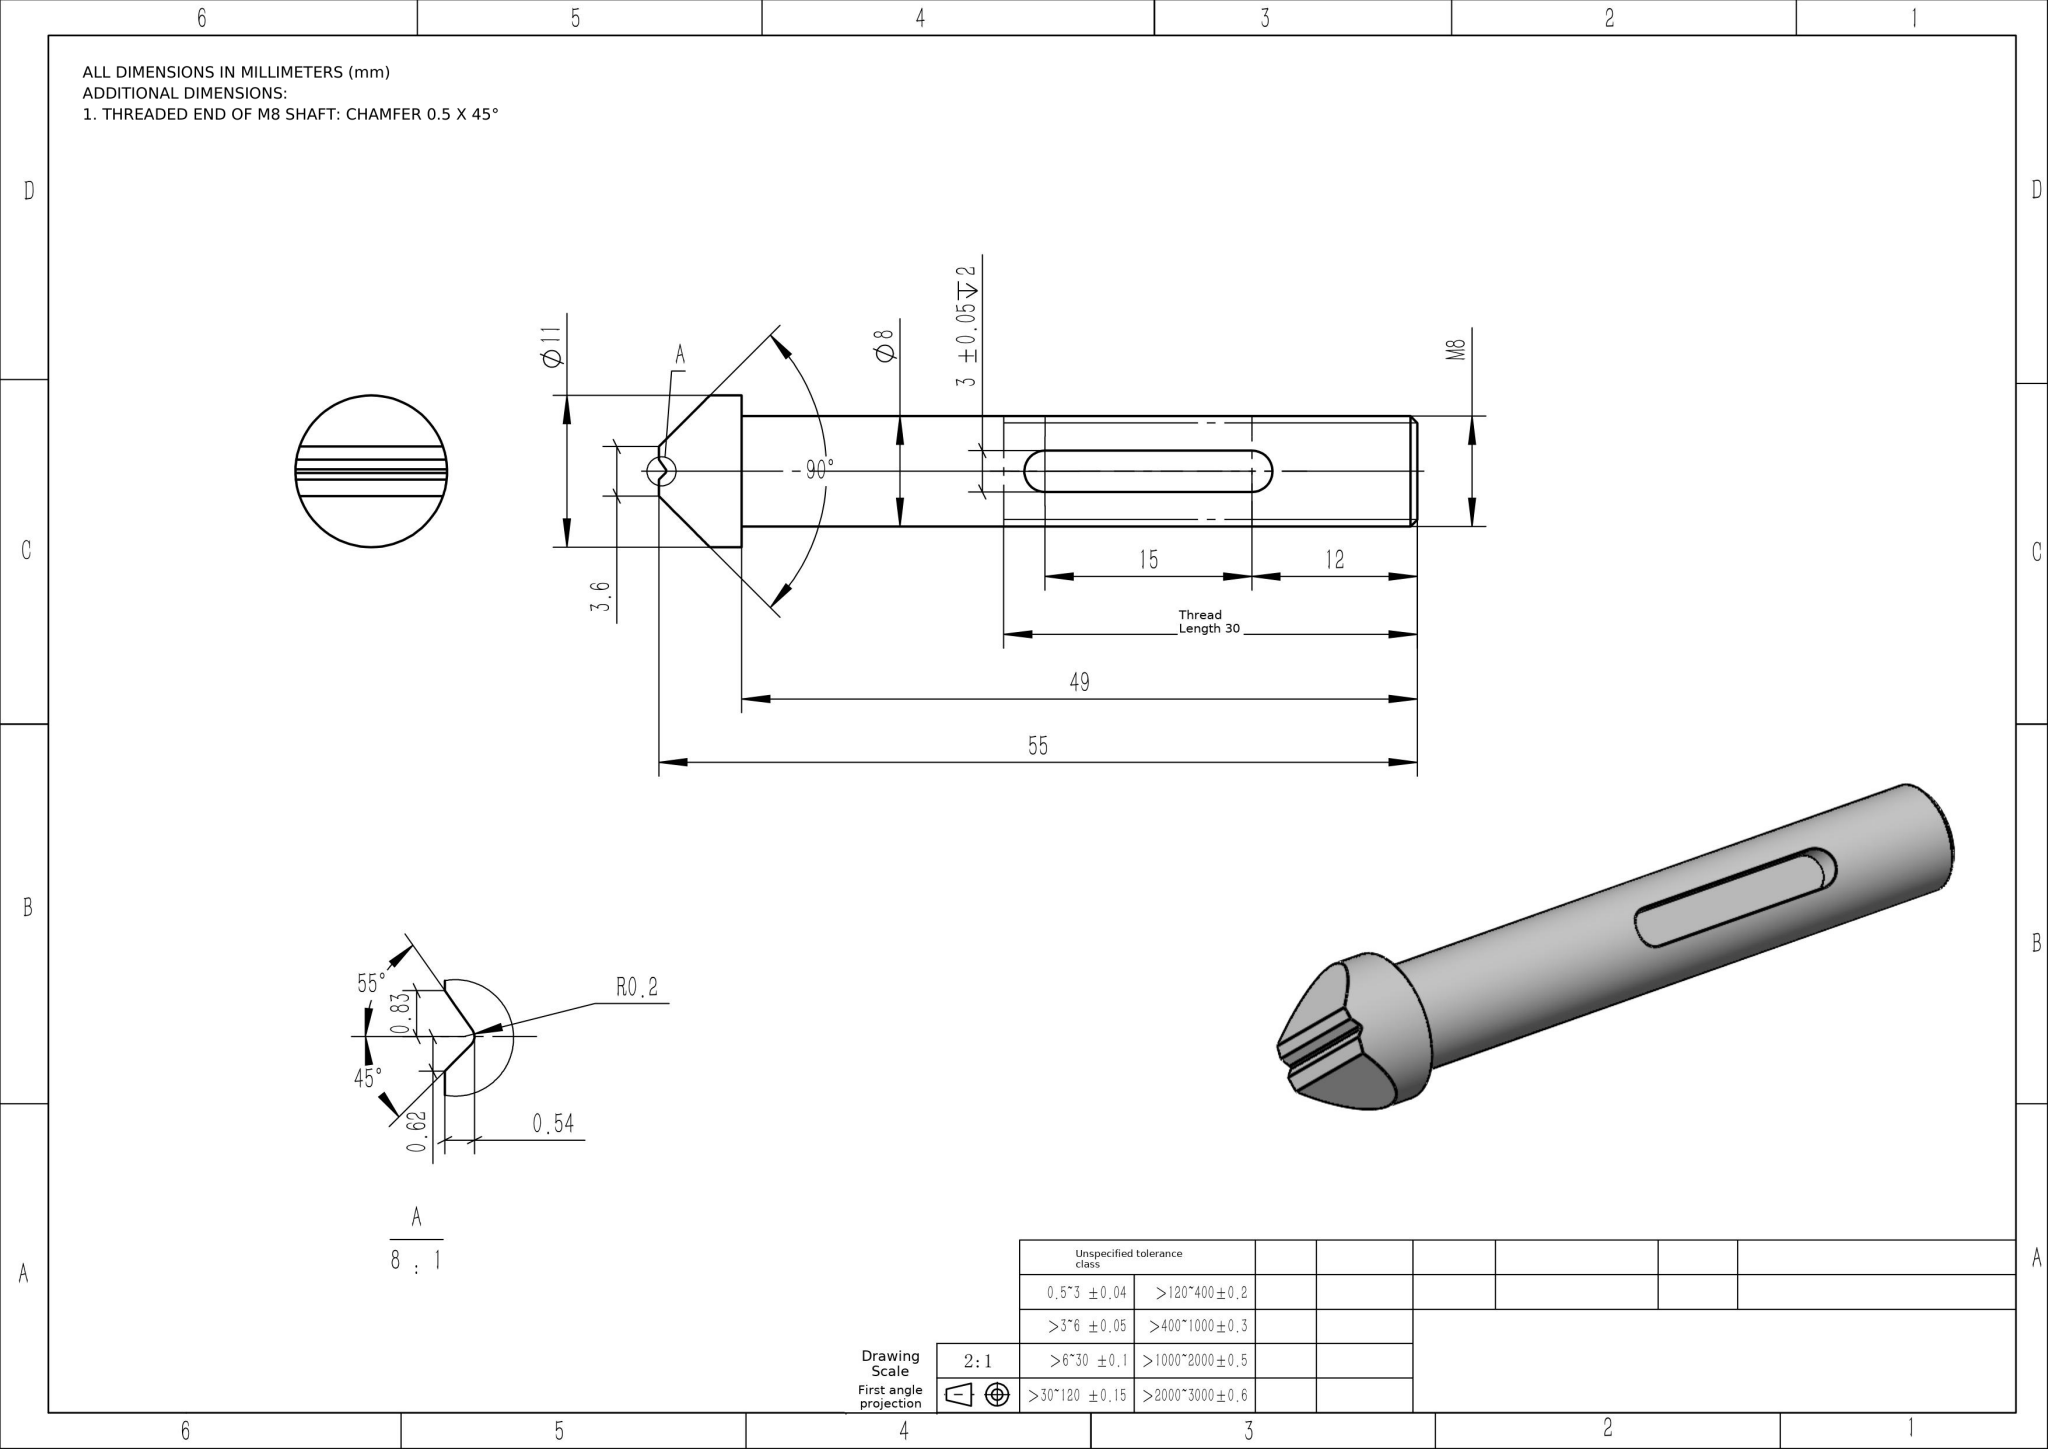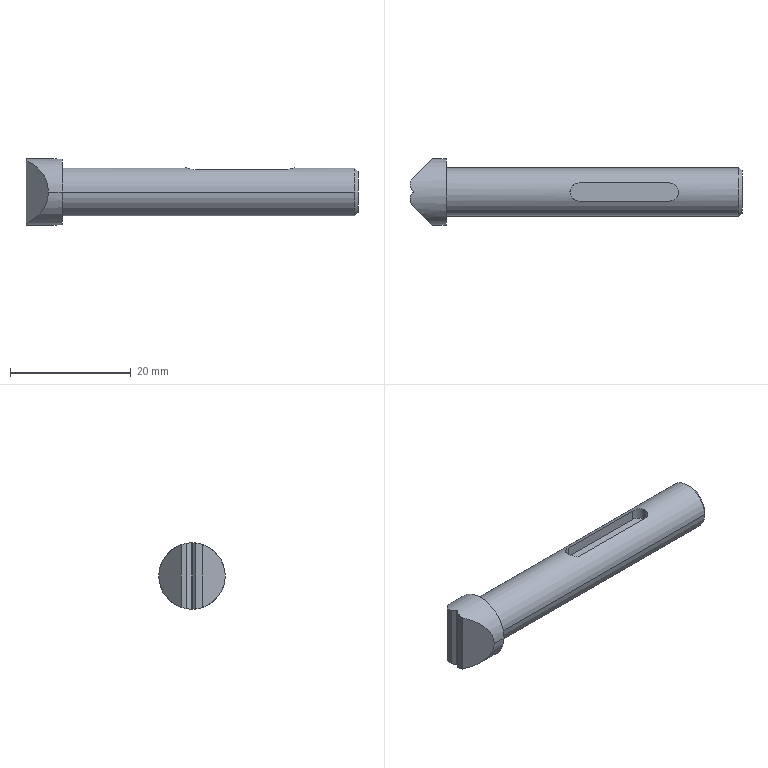Part | NX | mm | 1 solid | 22 faces | box 55 x 11 x 11 mm | volume 2840 mm3 | plane 11 | cylinder 9 | cone 2 | commonest cylinder face diameters 3 x3 0.4 x2 8 x2 11 x2
STEP:
#1=COLOUR_RGB('',0.698,0.698,0.698);
#2=FILL_AREA_STYLE_COLOUR('',#1);
#3=FILL_AREA_STYLE('',(#2));
#4=SURFACE_STYLE_FILL_AREA(#3);
#5=SURFACE_SIDE_STYLE('',(#4));
#6=SURFACE_STYLE_USAGE(.BOTH.,#5);
#7=PRESENTATION_STYLE_ASSIGNMENT((#6));
#8=CARTESIAN_POINT('',(44.5,0.,2.));
#9=VERTEX_POINT('',#8);
#10=CARTESIAN_POINT('',(43.,1.5,2.));
#11=VERTEX_POINT('',#10);
#12=CARTESIAN_POINT('',(43.,0.,2.));
#13=DIRECTION('',(0.,0.,1.));
#14=DIRECTION('',(1.,0.,0.));
#15=AXIS2_PLACEMENT_3D('',#12,#13,#14);
#16=CIRCLE('',#15,1.5);
#17=EDGE_CURVE('',#9,#11,#16,.T.);
#18=ORIENTED_EDGE('',*,*,#17,.F.);
#19=CARTESIAN_POINT('',(44.5,0.,4.));
#20=VERTEX_POINT('',#19);
#21=CARTESIAN_POINT('',(44.5,0.,2.));
#22=DIRECTION('',(0.,0.,1.));
#23=VECTOR('',#22,1000.);
#24=LINE('',#21,#23);
#25=EDGE_CURVE('',#9,#20,#24,.T.);
#26=ORIENTED_EDGE('',*,*,#25,.T.);
#27=CARTESIAN_POINT('',(43.,1.5,3.708));
#28=VERTEX_POINT('',#27);
#29=CARTESIAN_POINT('',(44.5,0.,4.));
#30=CARTESIAN_POINT('',(44.5,0.0988,4.));
#31=CARTESIAN_POINT('',(44.49,0.1991,3.996));
#32=CARTESIAN_POINT('',(44.451,0.3921,3.982));
#33=CARTESIAN_POINT('',(44.423,0.486,3.971));
#34=CARTESIAN_POINT('',(44.346,0.6687,3.945));
#35=CARTESIAN_POINT('',(44.3,0.7547,3.929));
#36=CARTESIAN_POINT('',(44.192,0.9162,3.895));
#37=CARTESIAN_POINT('',(44.129,0.9924,3.876));
#38=CARTESIAN_POINT('',(43.991,1.13,3.838));
#39=CARTESIAN_POINT('',(43.917,1.191,3.819));
#40=CARTESIAN_POINT('',(43.755,1.3,3.783));
#41=CARTESIAN_POINT('',(43.668,1.347,3.767));
#42=CARTESIAN_POINT('',(43.398,1.459,3.725));
#43=CARTESIAN_POINT('',(43.2,1.5,3.708));
#44=CARTESIAN_POINT('',(43.,1.5,3.708));
#45=B_SPLINE_CURVE_WITH_KNOTS('',3,(#29,#30,#31,#32,#33,#34,#35,#36,#37,#38,#39,#40,#41,#42,#43,#44),.UNSPECIFIED.,.F.,.F.,(4,2,2,2,2,2,2,4),(0.002367,0.002663,0.002958,0.003254,0.003549,0.003845,0.00414,0.004731),.UNSPECIFIED.);
#46=EDGE_CURVE('',#20,#28,#45,.T.);
#47=ORIENTED_EDGE('',*,*,#46,.T.);
#48=CARTESIAN_POINT('',(43.,1.5,2.));
#49=DIRECTION('',(0.,0.,1.));
#50=VECTOR('',#49,1000.);
#51=LINE('',#48,#50);
#52=EDGE_CURVE('',#11,#28,#51,.T.);
#53=ORIENTED_EDGE('',*,*,#52,.F.);
#54=EDGE_LOOP('',(#18,#26,#47,#53));
#55=FACE_OUTER_BOUND('',#54,.T.);
#56=CARTESIAN_POINT('',(43.,0.,2.));
#57=DIRECTION('',(0.,0.,1.));
#58=DIRECTION('',(1.,0.,0.));
#59=AXIS2_PLACEMENT_3D('',#56,#57,#58);
#60=CYLINDRICAL_SURFACE('',#59,1.5);
#61=ADVANCED_FACE('',(#55),#60,.F.);
#62=CARTESIAN_POINT('',(0.5037,0.1375,-5.498));
#63=VERTEX_POINT('',#62);
#64=CARTESIAN_POINT('',(0.5399,0.02275,-5.5));
#65=VERTEX_POINT('',#64);
#66=CARTESIAN_POINT('',(0.5037,0.1375,-5.498));
#67=CARTESIAN_POINT('',(0.5273,0.1038,-5.499));
#68=CARTESIAN_POINT('',(0.5399,0.06353,-5.5));
#69=CARTESIAN_POINT('',(0.5399,0.02275,-5.5));
#70=B_SPLINE_CURVE_WITH_KNOTS('',3,(#66,#67,#68,#69),.UNSPECIFIED.,.F.,.F.,(4,4),(0.,0.0001217),.UNSPECIFIED.);
#71=EDGE_CURVE('',#63,#65,#70,.T.);
#72=ORIENTED_EDGE('',*,*,#71,.T.);
#73=CARTESIAN_POINT('',(0.5399,0.02275,5.5));
#74=VERTEX_POINT('',#73);
#75=CARTESIAN_POINT('',(0.5399,0.02275,-10.));
#76=DIRECTION('',(0.,0.,1.));
#77=VECTOR('',#76,1000.);
#78=LINE('',#75,#77);
#79=EDGE_CURVE('',#65,#74,#78,.T.);
#80=ORIENTED_EDGE('',*,*,#79,.T.);
#81=CARTESIAN_POINT('',(0.5037,0.1375,5.498));
#82=VERTEX_POINT('',#81);
#83=CARTESIAN_POINT('',(0.5399,0.02275,5.5));
#84=CARTESIAN_POINT('',(0.5399,0.06334,5.5));
#85=CARTESIAN_POINT('',(0.5273,0.1038,5.499));
#86=CARTESIAN_POINT('',(0.5037,0.1375,5.498));
#87=B_SPLINE_CURVE_WITH_KNOTS('',3,(#83,#84,#85,#86),.UNSPECIFIED.,.F.,.F.,(4,4),(0.0001563,0.0002779),.UNSPECIFIED.);
#88=EDGE_CURVE('',#74,#82,#87,.T.);
#89=ORIENTED_EDGE('',*,*,#88,.T.);
#90=CARTESIAN_POINT('',(0.5037,0.1375,-10.));
#91=DIRECTION('',(0.,0.,1.));
#92=VECTOR('',#91,1000.);
#93=LINE('',#90,#92);
#94=EDGE_CURVE('',#63,#82,#93,.T.);
#95=ORIENTED_EDGE('',*,*,#94,.F.);
#96=EDGE_LOOP('',(#72,#80,#89,#95));
#97=FACE_OUTER_BOUND('',#96,.T.);
#98=CARTESIAN_POINT('',(0.3399,0.02275,-10.));
#99=DIRECTION('',(0.,0.,1.));
#100=DIRECTION('',(1.,0.,0.));
#101=AXIS2_PLACEMENT_3D('',#98,#99,#100);
#102=CYLINDRICAL_SURFACE('',#101,0.2);
#103=ADVANCED_FACE('',(#97),#102,.F.);
#104=CARTESIAN_POINT('',(55.,3.5,0.));
#105=VERTEX_POINT('',#104);
#106=CARTESIAN_POINT('',(55.,-3.5,0.));
#107=VERTEX_POINT('',#106);
#108=CARTESIAN_POINT('',(55.,-0.,0.));
#109=DIRECTION('',(1.,-0.,0.));
#110=DIRECTION('',(0.,1.,0.));
#111=AXIS2_PLACEMENT_3D('',#108,#109,#110);
#112=CIRCLE('',#111,3.5);
#113=EDGE_CURVE('',#105,#107,#112,.T.);
#114=ORIENTED_EDGE('',*,*,#113,.F.);
#115=CARTESIAN_POINT('',(54.5,4.,0.));
#116=VERTEX_POINT('',#115);
#117=CARTESIAN_POINT('',(55.,3.5,0.));
#118=DIRECTION('',(-0.7071,0.7071,0.));
#119=VECTOR('',#118,1000.);
#120=LINE('',#117,#119);
#121=EDGE_CURVE('',#105,#116,#120,.T.);
#122=ORIENTED_EDGE('',*,*,#121,.T.);
#123=CARTESIAN_POINT('',(54.5,-4.,0.));
#124=VERTEX_POINT('',#123);
#125=CARTESIAN_POINT('',(54.5,-0.,0.));
#126=DIRECTION('',(1.,-0.,0.));
#127=DIRECTION('',(0.,1.,0.));
#128=AXIS2_PLACEMENT_3D('',#125,#126,#127);
#129=CIRCLE('',#128,4.);
#130=EDGE_CURVE('',#116,#124,#129,.T.);
#131=ORIENTED_EDGE('',*,*,#130,.T.);
#132=CARTESIAN_POINT('',(55.,-3.5,0.));
#133=DIRECTION('',(-0.7071,-0.7071,0.));
#134=VECTOR('',#133,1000.);
#135=LINE('',#132,#134);
#136=EDGE_CURVE('',#107,#124,#135,.T.);
#137=ORIENTED_EDGE('',*,*,#136,.F.);
#138=EDGE_LOOP('',(#114,#122,#131,#137));
#139=FACE_OUTER_BOUND('',#138,.T.);
#140=CARTESIAN_POINT('',(55.,-0.,0.));
#141=DIRECTION('',(-1.,0.,0.));
#142=DIRECTION('',(0.,-1.,0.));
#143=AXIS2_PLACEMENT_3D('',#140,#141,#142);
#144=CONICAL_SURFACE('',#143,3.5,0.7854);
#145=ADVANCED_FACE('',(#139),#144,.T.);
#146=CARTESIAN_POINT('',(43.,-1.5,3.708));
#147=VERTEX_POINT('',#146);
#148=CARTESIAN_POINT('',(43.,-1.5,3.708));
#149=CARTESIAN_POINT('',(43.1,-1.5,3.708));
#150=CARTESIAN_POINT('',(43.198,-1.49,3.712));
#151=CARTESIAN_POINT('',(43.391,-1.451,3.727));
#152=CARTESIAN_POINT('',(43.487,-1.422,3.739));
#153=CARTESIAN_POINT('',(43.759,-1.309,3.781));
#154=CARTESIAN_POINT('',(43.924,-1.197,3.819));
#155=CARTESIAN_POINT('',(44.198,-0.9232,3.895));
#156=CARTESIAN_POINT('',(44.309,-0.7573,3.932));
#157=CARTESIAN_POINT('',(44.422,-0.4867,3.971));
#158=CARTESIAN_POINT('',(44.451,-0.3912,3.982));
#159=CARTESIAN_POINT('',(44.49,-0.197,3.996));
#160=CARTESIAN_POINT('',(44.5,-0.09895,4.));
#161=CARTESIAN_POINT('',(44.5,0.,4.));
#162=B_SPLINE_CURVE_WITH_KNOTS('',3,(#148,#149,#150,#151,#152,#153,#154,#155,#156,#157,#158,#159,#160,#161),.UNSPECIFIED.,.F.,.F.,(4,2,2,2,2,2,4),(0.,0.0002959,0.0005918,0.001184,0.001775,0.002071,0.002367),.UNSPECIFIED.);
#163=EDGE_CURVE('',#147,#20,#162,.T.);
#164=ORIENTED_EDGE('',*,*,#163,.F.);
#165=CARTESIAN_POINT('',(28.,-1.5,3.708));
#166=VERTEX_POINT('',#165);
#167=CARTESIAN_POINT('',(55.,-1.5,3.708));
#168=DIRECTION('',(1.,-0.,0.));
#169=VECTOR('',#168,1000.);
#170=LINE('',#167,#169);
#171=EDGE_CURVE('',#166,#147,#170,.T.);
#172=ORIENTED_EDGE('',*,*,#171,.F.);
#173=CARTESIAN_POINT('',(28.,1.5,3.708));
#174=VERTEX_POINT('',#173);
#175=CARTESIAN_POINT('',(28.,1.5,3.708));
#176=CARTESIAN_POINT('',(27.9,1.5,3.708));
#177=CARTESIAN_POINT('',(27.802,1.49,3.712));
#178=CARTESIAN_POINT('',(27.609,1.451,3.727));
#179=CARTESIAN_POINT('',(27.513,1.422,3.739));
#180=CARTESIAN_POINT('',(27.242,1.309,3.781));
#181=CARTESIAN_POINT('',(27.077,1.198,3.819));
#182=CARTESIAN_POINT('',(26.803,0.924,3.894));
#183=CARTESIAN_POINT('',(26.691,0.7582,3.932));
#184=CARTESIAN_POINT('',(26.578,0.488,3.971));
#185=CARTESIAN_POINT('',(26.549,0.3926,3.982));
#186=CARTESIAN_POINT('',(26.51,0.1986,3.996));
#187=CARTESIAN_POINT('',(26.5,0.1006,4.));
#188=CARTESIAN_POINT('',(26.5,-0.09712,4.));
#189=CARTESIAN_POINT('',(26.51,-0.1975,3.996));
#190=CARTESIAN_POINT('',(26.548,-0.3907,3.982));
#191=CARTESIAN_POINT('',(26.577,-0.4847,3.972));
#192=CARTESIAN_POINT('',(26.691,-0.759,3.932));
#193=CARTESIAN_POINT('',(26.802,-0.9229,3.895));
#194=CARTESIAN_POINT('',(27.008,-1.129,3.838));
#195=CARTESIAN_POINT('',(27.083,-1.191,3.819));
#196=CARTESIAN_POINT('',(27.244,-1.299,3.783));
#197=CARTESIAN_POINT('',(27.332,-1.347,3.767));
#198=CARTESIAN_POINT('',(27.602,-1.459,3.725));
#199=CARTESIAN_POINT('',(27.8,-1.5,3.708));
#200=CARTESIAN_POINT('',(28.,-1.5,3.708));
#201=B_SPLINE_CURVE_WITH_KNOTS('',3,(#175,#176,#177,#178,#179,#180,#181,#182,#183,#184,#185,#186,#187,#188,#189,#190,#191,#192,#193,#194,#195,#196,#197,#198,#199,#200),.UNSPECIFIED.,.F.,.F.,(4,2,2,2,2,2,2,2,2,2,2,2,4),(0.,0.0002957,0.0005914,0.001183,0.001774,0.00207,0.002366,0.002661,0.002957,0.003548,0.003844,0.00414,0.004731),.UNSPECIFIED.);
#202=EDGE_CURVE('',#174,#166,#201,.T.);
#203=ORIENTED_EDGE('',*,*,#202,.F.);
#204=CARTESIAN_POINT('',(55.,1.5,3.708));
#205=DIRECTION('',(-1.,0.,0.));
#206=VECTOR('',#205,1000.);
#207=LINE('',#204,#206);
#208=EDGE_CURVE('',#28,#174,#207,.T.);
#209=ORIENTED_EDGE('',*,*,#208,.F.);
#210=ORIENTED_EDGE('',*,*,#46,.F.);
#211=EDGE_LOOP('',(#164,#172,#203,#209,#210));
#212=FACE_BOUND('',#211,.T.);
#213=CARTESIAN_POINT('',(6.,4.,0.));
#214=VERTEX_POINT('',#213);
#215=CARTESIAN_POINT('',(6.,-4.,0.));
#216=VERTEX_POINT('',#215);
#217=CARTESIAN_POINT('',(6.,-0.,0.));
#218=DIRECTION('',(1.,-0.,0.));
#219=DIRECTION('',(0.,1.,0.));
#220=AXIS2_PLACEMENT_3D('',#217,#218,#219);
#221=CIRCLE('',#220,4.);
#222=EDGE_CURVE('',#214,#216,#221,.T.);
#223=ORIENTED_EDGE('',*,*,#222,.T.);
#224=CARTESIAN_POINT('',(55.,-4.,0.));
#225=DIRECTION('',(1.,-0.,0.));
#226=VECTOR('',#225,1000.);
#227=LINE('',#224,#226);
#228=EDGE_CURVE('',#216,#124,#227,.T.);
#229=ORIENTED_EDGE('',*,*,#228,.T.);
#230=ORIENTED_EDGE('',*,*,#130,.F.);
#231=CARTESIAN_POINT('',(55.,4.,0.));
#232=DIRECTION('',(1.,-0.,0.));
#233=VECTOR('',#232,1000.);
#234=LINE('',#231,#233);
#235=EDGE_CURVE('',#214,#116,#234,.T.);
#236=ORIENTED_EDGE('',*,*,#235,.F.);
#237=EDGE_LOOP('',(#223,#229,#230,#236));
#238=FACE_OUTER_BOUND('',#237,.T.);
#239=CARTESIAN_POINT('',(55.,-0.,0.));
#240=DIRECTION('',(1.,-0.,0.));
#241=DIRECTION('',(0.,1.,0.));
#242=AXIS2_PLACEMENT_3D('',#239,#240,#241);
#243=CYLINDRICAL_SURFACE('',#242,4.);
#244=ADVANCED_FACE('',(#212,#238),#243,.T.);
#245=CARTESIAN_POINT('',(3.7,-5.5,0.));
#246=VERTEX_POINT('',#245);
#247=CARTESIAN_POINT('',(0.,-1.8,5.197));
#248=VERTEX_POINT('',#247);
#249=CARTESIAN_POINT('',(3.7,-5.5,0.));
#250=CARTESIAN_POINT('',(3.7,-5.5,2.426));
#251=CARTESIAN_POINT('',(2.293,-4.093,4.403));
#252=CARTESIAN_POINT('',(0.,-1.8,5.197));
#253=(BOUNDED_CURVE()B_SPLINE_CURVE(3,(#249,#250,#251,#252),.UNSPECIFIED.,.F.,.F.)B_SPLINE_CURVE_WITH_KNOTS((4,4),(0.,1.237),.UNSPECIFIED.)CURVE()GEOMETRIC_REPRESENTATION_ITEM()RATIONAL_B_SPLINE_CURVE((1.,0.8764,0.8764,1.))REPRESENTATION_ITEM(''));
#254=EDGE_CURVE('',#246,#248,#253,.T.);
#255=ORIENTED_EDGE('',*,*,#254,.F.);
#256=CARTESIAN_POINT('',(6.,-5.5,0.));
#257=VERTEX_POINT('',#256);
#258=CARTESIAN_POINT('',(55.,-5.5,0.));
#259=DIRECTION('',(1.,-0.,0.));
#260=VECTOR('',#259,1000.);
#261=LINE('',#258,#260);
#262=EDGE_CURVE('',#246,#257,#261,.T.);
#263=ORIENTED_EDGE('',*,*,#262,.T.);
#264=CARTESIAN_POINT('',(6.,5.5,0.));
#265=VERTEX_POINT('',#264);
#266=CARTESIAN_POINT('',(6.,-0.,0.));
#267=DIRECTION('',(1.,-0.,0.));
#268=DIRECTION('',(0.,1.,0.));
#269=AXIS2_PLACEMENT_3D('',#266,#267,#268);
#270=CIRCLE('',#269,5.5);
#271=EDGE_CURVE('',#265,#257,#270,.T.);
#272=ORIENTED_EDGE('',*,*,#271,.F.);
#273=CARTESIAN_POINT('',(3.7,5.5,0.));
#274=VERTEX_POINT('',#273);
#275=CARTESIAN_POINT('',(55.,5.5,0.));
#276=DIRECTION('',(1.,-0.,0.));
#277=VECTOR('',#276,1000.);
#278=LINE('',#275,#277);
#279=EDGE_CURVE('',#274,#265,#278,.T.);
#280=ORIENTED_EDGE('',*,*,#279,.F.);
#281=CARTESIAN_POINT('',(0.,1.8,5.197));
#282=VERTEX_POINT('',#281);
#283=CARTESIAN_POINT('',(0.,1.8,5.197));
#284=CARTESIAN_POINT('',(2.293,4.093,4.403));
#285=CARTESIAN_POINT('',(3.7,5.5,2.426));
#286=CARTESIAN_POINT('',(3.7,5.5,0.));
#287=(BOUNDED_CURVE()B_SPLINE_CURVE(3,(#283,#284,#285,#286),.UNSPECIFIED.,.F.,.T.)B_SPLINE_CURVE_WITH_KNOTS((4,4),(5.046,6.283),.UNSPECIFIED.)CURVE()GEOMETRIC_REPRESENTATION_ITEM()RATIONAL_B_SPLINE_CURVE((1.,0.8764,0.8764,1.))REPRESENTATION_ITEM(''));
#288=EDGE_CURVE('',#282,#274,#287,.T.);
#289=ORIENTED_EDGE('',*,*,#288,.F.);
#290=CARTESIAN_POINT('',(0.,0.8569,5.433));
#291=VERTEX_POINT('',#290);
#292=CARTESIAN_POINT('',(0.,0.,0.));
#293=DIRECTION('',(1.,-0.,0.));
#294=DIRECTION('',(0.,1.,0.));
#295=AXIS2_PLACEMENT_3D('',#292,#293,#294);
#296=CIRCLE('',#295,5.5);
#297=EDGE_CURVE('',#282,#291,#296,.T.);
#298=ORIENTED_EDGE('',*,*,#297,.T.);
#299=CARTESIAN_POINT('',(0.5037,0.1375,5.498));
#300=CARTESIAN_POINT('',(0.3349,0.3785,5.492));
#301=CARTESIAN_POINT('',(0.1668,0.6187,5.47));
#302=CARTESIAN_POINT('',(0.,0.8569,5.433));
#303=(BOUNDED_CURVE()B_SPLINE_CURVE(3,(#299,#300,#301,#302),.UNSPECIFIED.,.F.,.T.)B_SPLINE_CURVE_WITH_KNOTS((4,4),(1.596,1.727),.UNSPECIFIED.)CURVE()GEOMETRIC_REPRESENTATION_ITEM()RATIONAL_B_SPLINE_CURVE((1.,0.9986,0.9986,1.))REPRESENTATION_ITEM(''));
#304=EDGE_CURVE('',#82,#291,#303,.T.);
#305=ORIENTED_EDGE('',*,*,#304,.F.);
#306=ORIENTED_EDGE('',*,*,#88,.F.);
#307=CARTESIAN_POINT('',(0.4813,-0.1187,5.499));
#308=VERTEX_POINT('',#307);
#309=CARTESIAN_POINT('',(0.4813,-0.1187,5.499));
#310=CARTESIAN_POINT('',(0.5187,-0.0813,5.5));
#311=CARTESIAN_POINT('',(0.5399,-0.02943,5.5));
#312=CARTESIAN_POINT('',(0.5399,0.02275,5.5));
#313=B_SPLINE_CURVE_WITH_KNOTS('',3,(#309,#310,#311,#312),.UNSPECIFIED.,.F.,.F.,(4,4),(0.,0.0001563),.UNSPECIFIED.);
#314=EDGE_CURVE('',#308,#74,#313,.T.);
#315=ORIENTED_EDGE('',*,*,#314,.F.);
#316=CARTESIAN_POINT('',(0.,-0.6,5.467));
#317=VERTEX_POINT('',#316);
#318=CARTESIAN_POINT('',(0.,-0.6,5.467));
#319=CARTESIAN_POINT('',(0.1599,-0.4401,5.485));
#320=CARTESIAN_POINT('',(0.3205,-0.2795,5.495));
#321=CARTESIAN_POINT('',(0.4813,-0.1187,5.499));
#322=(BOUNDED_CURVE()B_SPLINE_CURVE(3,(#318,#319,#320,#321),.UNSPECIFIED.,.F.,.F.)B_SPLINE_CURVE_WITH_KNOTS((4,4),(4.603,4.691),.UNSPECIFIED.)CURVE()GEOMETRIC_REPRESENTATION_ITEM()RATIONAL_B_SPLINE_CURVE((1.,0.9994,0.9994,1.))REPRESENTATION_ITEM(''));
#323=EDGE_CURVE('',#317,#308,#322,.T.);
#324=ORIENTED_EDGE('',*,*,#323,.F.);
#325=CARTESIAN_POINT('',(0.,0.,0.));
#326=DIRECTION('',(1.,-0.,0.));
#327=DIRECTION('',(0.,1.,0.));
#328=AXIS2_PLACEMENT_3D('',#325,#326,#327);
#329=CIRCLE('',#328,5.5);
#330=EDGE_CURVE('',#317,#248,#329,.T.);
#331=ORIENTED_EDGE('',*,*,#330,.T.);
#332=EDGE_LOOP('',(#255,#263,#272,#280,#289,#298,#305,#306,#315,#324,#331));
#333=FACE_OUTER_BOUND('',#332,.T.);
#334=CARTESIAN_POINT('',(55.,-0.,0.));
#335=DIRECTION('',(1.,-0.,0.));
#336=DIRECTION('',(0.,1.,0.));
#337=AXIS2_PLACEMENT_3D('',#334,#335,#336);
#338=CYLINDRICAL_SURFACE('',#337,5.5);
#339=ADVANCED_FACE('',(#333),#338,.T.);
#340=CARTESIAN_POINT('',(0.,1.8,-5.197));
#341=VERTEX_POINT('',#340);
#342=CARTESIAN_POINT('',(0.,1.8,-10.));
#343=DIRECTION('',(0.,0.,1.));
#344=VECTOR('',#343,1000.);
#345=LINE('',#342,#344);
#346=EDGE_CURVE('',#341,#282,#345,.T.);
#347=ORIENTED_EDGE('',*,*,#346,.F.);
#348=CARTESIAN_POINT('',(0.,0.8569,-5.433));
#349=VERTEX_POINT('',#348);
#350=CARTESIAN_POINT('',(0.,0.,0.));
#351=DIRECTION('',(1.,-0.,0.));
#352=DIRECTION('',(0.,1.,0.));
#353=AXIS2_PLACEMENT_3D('',#350,#351,#352);
#354=CIRCLE('',#353,5.5);
#355=EDGE_CURVE('',#349,#341,#354,.T.);
#356=ORIENTED_EDGE('',*,*,#355,.F.);
#357=CARTESIAN_POINT('',(0.,0.8569,-10.));
#358=DIRECTION('',(0.,0.,1.));
#359=VECTOR('',#358,1000.);
#360=LINE('',#357,#359);
#361=EDGE_CURVE('',#349,#291,#360,.T.);
#362=ORIENTED_EDGE('',*,*,#361,.T.);
#363=ORIENTED_EDGE('',*,*,#297,.F.);
#364=EDGE_LOOP('',(#347,#356,#362,#363));
#365=FACE_OUTER_BOUND('',#364,.T.);
#366=CARTESIAN_POINT('',(0.,0.,0.));
#367=DIRECTION('',(-1.,0.,0.));
#368=DIRECTION('',(-0.,-1.,0.));
#369=AXIS2_PLACEMENT_3D('',#366,#367,#368);
#370=PLANE('',#369);
#371=ADVANCED_FACE('',(#365),#370,.T.);
#372=CARTESIAN_POINT('',(0.,-1.8,-5.197));
#373=VERTEX_POINT('',#372);
#374=CARTESIAN_POINT('',(0.,-1.8,-10.));
#375=DIRECTION('',(0.,0.,1.));
#376=VECTOR('',#375,1000.);
#377=LINE('',#374,#376);
#378=EDGE_CURVE('',#373,#248,#377,.T.);
#379=ORIENTED_EDGE('',*,*,#378,.T.);
#380=ORIENTED_EDGE('',*,*,#330,.F.);
#381=CARTESIAN_POINT('',(0.,-0.6,-5.467));
#382=VERTEX_POINT('',#381);
#383=CARTESIAN_POINT('',(0.,-0.6,-10.));
#384=DIRECTION('',(0.,0.,1.));
#385=VECTOR('',#384,1000.);
#386=LINE('',#383,#385);
#387=EDGE_CURVE('',#382,#317,#386,.T.);
#388=ORIENTED_EDGE('',*,*,#387,.F.);
#389=CARTESIAN_POINT('',(0.,0.,0.));
#390=DIRECTION('',(1.,-0.,0.));
#391=DIRECTION('',(0.,1.,0.));
#392=AXIS2_PLACEMENT_3D('',#389,#390,#391);
#393=CIRCLE('',#392,5.5);
#394=EDGE_CURVE('',#373,#382,#393,.T.);
#395=ORIENTED_EDGE('',*,*,#394,.F.);
#396=EDGE_LOOP('',(#379,#380,#388,#395));
#397=FACE_OUTER_BOUND('',#396,.T.);
#398=CARTESIAN_POINT('',(0.,0.,0.));
#399=DIRECTION('',(-1.,0.,0.));
#400=DIRECTION('',(-0.,-1.,0.));
#401=AXIS2_PLACEMENT_3D('',#398,#399,#400);
#402=PLANE('',#401);
#403=ADVANCED_FACE('',(#397),#402,.T.);
#404=ORIENTED_EDGE('',*,*,#262,.F.);
#405=CARTESIAN_POINT('',(0.,-1.8,-5.197));
#406=CARTESIAN_POINT('',(2.293,-4.093,-4.403));
#407=CARTESIAN_POINT('',(3.7,-5.5,-2.426));
#408=CARTESIAN_POINT('',(3.7,-5.5,0.));
#409=(BOUNDED_CURVE()B_SPLINE_CURVE(3,(#405,#406,#407,#408),.UNSPECIFIED.,.F.,.F.)B_SPLINE_CURVE_WITH_KNOTS((4,4),(5.046,6.283),.UNSPECIFIED.)CURVE()GEOMETRIC_REPRESENTATION_ITEM()RATIONAL_B_SPLINE_CURVE((1.,0.8764,0.8764,1.))REPRESENTATION_ITEM(''));
#410=EDGE_CURVE('',#373,#246,#409,.T.);
#411=ORIENTED_EDGE('',*,*,#410,.F.);
#412=ORIENTED_EDGE('',*,*,#394,.T.);
#413=CARTESIAN_POINT('',(0.4813,-0.1187,-5.499));
#414=VERTEX_POINT('',#413);
#415=CARTESIAN_POINT('',(0.4813,-0.1187,-5.499));
#416=CARTESIAN_POINT('',(0.3205,-0.2795,-5.495));
#417=CARTESIAN_POINT('',(0.1599,-0.4401,-5.485));
#418=CARTESIAN_POINT('',(0.,-0.6,-5.467));
#419=(BOUNDED_CURVE()B_SPLINE_CURVE(3,(#415,#416,#417,#418),.UNSPECIFIED.,.F.,.T.)B_SPLINE_CURVE_WITH_KNOTS((4,4),(1.592,1.68),.UNSPECIFIED.)CURVE()GEOMETRIC_REPRESENTATION_ITEM()RATIONAL_B_SPLINE_CURVE((1.,0.9994,0.9994,1.))REPRESENTATION_ITEM(''));
#420=EDGE_CURVE('',#414,#382,#419,.T.);
#421=ORIENTED_EDGE('',*,*,#420,.F.);
#422=CARTESIAN_POINT('',(0.5399,0.02275,-5.5));
#423=CARTESIAN_POINT('',(0.5399,-0.0296,-5.5));
#424=CARTESIAN_POINT('',(0.5187,-0.08133,-5.5));
#425=CARTESIAN_POINT('',(0.4813,-0.1187,-5.499));
#426=B_SPLINE_CURVE_WITH_KNOTS('',3,(#422,#423,#424,#425),.UNSPECIFIED.,.F.,.F.,(4,4),(0.0001217,0.0002779),.UNSPECIFIED.);
#427=EDGE_CURVE('',#65,#414,#426,.T.);
#428=ORIENTED_EDGE('',*,*,#427,.F.);
#429=ORIENTED_EDGE('',*,*,#71,.F.);
#430=CARTESIAN_POINT('',(0.,0.8569,-5.433));
#431=CARTESIAN_POINT('',(0.1668,0.6187,-5.47));
#432=CARTESIAN_POINT('',(0.3349,0.3785,-5.492));
#433=CARTESIAN_POINT('',(0.5037,0.1375,-5.498));
#434=(BOUNDED_CURVE()B_SPLINE_CURVE(3,(#430,#431,#432,#433),.UNSPECIFIED.,.F.,.T.)B_SPLINE_CURVE_WITH_KNOTS((4,4),(4.556,4.687),.UNSPECIFIED.)CURVE()GEOMETRIC_REPRESENTATION_ITEM()RATIONAL_B_SPLINE_CURVE((1.,0.9986,0.9986,1.))REPRESENTATION_ITEM(''));
#435=EDGE_CURVE('',#349,#63,#434,.T.);
#436=ORIENTED_EDGE('',*,*,#435,.F.);
#437=ORIENTED_EDGE('',*,*,#355,.T.);
#438=CARTESIAN_POINT('',(3.7,5.5,0.));
#439=CARTESIAN_POINT('',(3.7,5.5,-2.426));
#440=CARTESIAN_POINT('',(2.293,4.093,-4.403));
#441=CARTESIAN_POINT('',(0.,1.8,-5.197));
#442=(BOUNDED_CURVE()B_SPLINE_CURVE(3,(#438,#439,#440,#441),.UNSPECIFIED.,.F.,.F.)B_SPLINE_CURVE_WITH_KNOTS((4,4),(0.,1.237),.UNSPECIFIED.)CURVE()GEOMETRIC_REPRESENTATION_ITEM()RATIONAL_B_SPLINE_CURVE((1.,0.8764,0.8764,1.))REPRESENTATION_ITEM(''));
#443=EDGE_CURVE('',#274,#341,#442,.T.);
#444=ORIENTED_EDGE('',*,*,#443,.F.);
#445=ORIENTED_EDGE('',*,*,#279,.T.);
#446=CARTESIAN_POINT('',(6.,-0.,0.));
#447=DIRECTION('',(1.,-0.,0.));
#448=DIRECTION('',(0.,1.,0.));
#449=AXIS2_PLACEMENT_3D('',#446,#447,#448);
#450=CIRCLE('',#449,5.5);
#451=EDGE_CURVE('',#257,#265,#450,.T.);
#452=ORIENTED_EDGE('',*,*,#451,.F.);
#453=EDGE_LOOP('',(#404,#411,#412,#421,#428,#429,#436,#437,#444,#445,#452));
#454=FACE_OUTER_BOUND('',#453,.T.);
#455=CARTESIAN_POINT('',(55.,-0.,0.));
#456=DIRECTION('',(1.,-0.,0.));
#457=DIRECTION('',(0.,1.,0.));
#458=AXIS2_PLACEMENT_3D('',#455,#456,#457);
#459=CYLINDRICAL_SURFACE('',#458,5.5);
#460=ADVANCED_FACE('',(#454),#459,.T.);
#461=ORIENTED_EDGE('',*,*,#271,.T.);
#462=ORIENTED_EDGE('',*,*,#451,.T.);
#463=EDGE_LOOP('',(#461,#462));
#464=FACE_OUTER_BOUND('',#463,.T.);
#465=ORIENTED_EDGE('',*,*,#222,.F.);
#466=CARTESIAN_POINT('',(6.,-0.,0.));
#467=DIRECTION('',(1.,-0.,0.));
#468=DIRECTION('',(0.,1.,0.));
#469=AXIS2_PLACEMENT_3D('',#466,#467,#468);
#470=CIRCLE('',#469,4.);
#471=EDGE_CURVE('',#216,#214,#470,.T.);
#472=ORIENTED_EDGE('',*,*,#471,.F.);
#473=EDGE_LOOP('',(#465,#472));
#474=FACE_BOUND('',#473,.T.);
#475=CARTESIAN_POINT('',(6.,5.5,0.));
#476=DIRECTION('',(1.,-0.,0.));
#477=DIRECTION('',(0.,1.,0.));
#478=AXIS2_PLACEMENT_3D('',#475,#476,#477);
#479=PLANE('',#478);
#480=ADVANCED_FACE('',(#464,#474),#479,.T.);
#481=ORIENTED_EDGE('',*,*,#228,.F.);
#482=ORIENTED_EDGE('',*,*,#471,.T.);
#483=ORIENTED_EDGE('',*,*,#235,.T.);
#484=CARTESIAN_POINT('',(54.5,-0.,0.));
#485=DIRECTION('',(1.,-0.,0.));
#486=DIRECTION('',(0.,1.,0.));
#487=AXIS2_PLACEMENT_3D('',#484,#485,#486);
#488=CIRCLE('',#487,4.);
#489=EDGE_CURVE('',#124,#116,#488,.T.);
#490=ORIENTED_EDGE('',*,*,#489,.F.);
#491=EDGE_LOOP('',(#481,#482,#483,#490));
#492=FACE_OUTER_BOUND('',#491,.T.);
#493=CARTESIAN_POINT('',(55.,-0.,0.));
#494=DIRECTION('',(1.,-0.,0.));
#495=DIRECTION('',(0.,1.,0.));
#496=AXIS2_PLACEMENT_3D('',#493,#494,#495);
#497=CYLINDRICAL_SURFACE('',#496,4.);
#498=ADVANCED_FACE('',(#492),#497,.T.);
#499=ORIENTED_EDGE('',*,*,#121,.F.);
#500=CARTESIAN_POINT('',(55.,-0.,0.));
#501=DIRECTION('',(1.,-0.,0.));
#502=DIRECTION('',(0.,1.,0.));
#503=AXIS2_PLACEMENT_3D('',#500,#501,#502);
#504=CIRCLE('',#503,3.5);
#505=EDGE_CURVE('',#107,#105,#504,.T.);
#506=ORIENTED_EDGE('',*,*,#505,.F.);
#507=ORIENTED_EDGE('',*,*,#136,.T.);
#508=ORIENTED_EDGE('',*,*,#489,.T.);
#509=EDGE_LOOP('',(#499,#506,#507,#508));
#510=FACE_OUTER_BOUND('',#509,.T.);
#511=CARTESIAN_POINT('',(55.,-0.,0.));
#512=DIRECTION('',(-1.,0.,0.));
#513=DIRECTION('',(0.,-1.,0.));
#514=AXIS2_PLACEMENT_3D('',#511,#512,#513);
#515=CONICAL_SURFACE('',#514,3.5,0.7854);
#516=ADVANCED_FACE('',(#510),#515,.T.);
#517=ORIENTED_EDGE('',*,*,#505,.T.);
#518=ORIENTED_EDGE('',*,*,#113,.T.);
#519=EDGE_LOOP('',(#517,#518));
#520=FACE_OUTER_BOUND('',#519,.T.);
#521=CARTESIAN_POINT('',(55.,3.5,0.));
#522=DIRECTION('',(1.,-0.,0.));
#523=DIRECTION('',(0.,1.,0.));
#524=AXIS2_PLACEMENT_3D('',#521,#522,#523);
#525=PLANE('',#524);
#526=ADVANCED_FACE('',(#520),#525,.T.);
#527=ORIENTED_EDGE('',*,*,#304,.T.);
#528=ORIENTED_EDGE('',*,*,#361,.F.);
#529=ORIENTED_EDGE('',*,*,#435,.T.);
#530=ORIENTED_EDGE('',*,*,#94,.T.);
#531=EDGE_LOOP('',(#527,#528,#529,#530));
#532=FACE_OUTER_BOUND('',#531,.T.);
#533=CARTESIAN_POINT('',(0.,0.8569,-10.));
#534=DIRECTION('',(0.8192,0.5736,0.));
#535=DIRECTION('',(-0.5736,0.8192,0.));
#536=AXIS2_PLACEMENT_3D('',#533,#534,#535);
#537=PLANE('',#536);
#538=ADVANCED_FACE('',(#532),#537,.F.);
#539=ORIENTED_EDGE('',*,*,#79,.F.);
#540=ORIENTED_EDGE('',*,*,#427,.T.);
#541=CARTESIAN_POINT('',(0.4813,-0.1187,-10.));
#542=DIRECTION('',(0.,0.,1.));
#543=VECTOR('',#542,1000.);
#544=LINE('',#541,#543);
#545=EDGE_CURVE('',#414,#308,#544,.T.);
#546=ORIENTED_EDGE('',*,*,#545,.T.);
#547=ORIENTED_EDGE('',*,*,#314,.T.);
#548=EDGE_LOOP('',(#539,#540,#546,#547));
#549=FACE_OUTER_BOUND('',#548,.T.);
#550=CARTESIAN_POINT('',(0.3399,0.02275,-10.));
#551=DIRECTION('',(0.,0.,1.));
#552=DIRECTION('',(1.,0.,0.));
#553=AXIS2_PLACEMENT_3D('',#550,#551,#552);
#554=CYLINDRICAL_SURFACE('',#553,0.2);
#555=ADVANCED_FACE('',(#549),#554,.F.);
#556=ORIENTED_EDGE('',*,*,#420,.T.);
#557=ORIENTED_EDGE('',*,*,#387,.T.);
#558=ORIENTED_EDGE('',*,*,#323,.T.);
#559=ORIENTED_EDGE('',*,*,#545,.F.);
#560=EDGE_LOOP('',(#556,#557,#558,#559));
#561=FACE_OUTER_BOUND('',#560,.T.);
#562=CARTESIAN_POINT('',(0.4813,-0.1187,-10.));
#563=DIRECTION('',(0.7071,-0.7071,0.));
#564=DIRECTION('',(0.7071,0.7071,0.));
#565=AXIS2_PLACEMENT_3D('',#562,#563,#564);
#566=PLANE('',#565);
#567=ADVANCED_FACE('',(#561),#566,.F.);
#568=ORIENTED_EDGE('',*,*,#288,.T.);
#569=ORIENTED_EDGE('',*,*,#443,.T.);
#570=ORIENTED_EDGE('',*,*,#346,.T.);
#571=EDGE_LOOP('',(#568,#569,#570));
#572=FACE_OUTER_BOUND('',#571,.T.);
#573=CARTESIAN_POINT('',(0.,1.8,-10.));
#574=DIRECTION('',(0.7071,-0.7071,0.));
#575=DIRECTION('',(0.7071,0.7071,0.));
#576=AXIS2_PLACEMENT_3D('',#573,#574,#575);
#577=PLANE('',#576);
#578=ADVANCED_FACE('',(#572),#577,.F.);
#579=ORIENTED_EDGE('',*,*,#410,.T.);
#580=ORIENTED_EDGE('',*,*,#254,.T.);
#581=ORIENTED_EDGE('',*,*,#378,.F.);
#582=EDGE_LOOP('',(#579,#580,#581));
#583=FACE_OUTER_BOUND('',#582,.T.);
#584=CARTESIAN_POINT('',(0.,-1.8,-10.));
#585=DIRECTION('',(0.7071,0.7071,0.));
#586=DIRECTION('',(-0.7071,0.7071,0.));
#587=AXIS2_PLACEMENT_3D('',#584,#585,#586);
#588=PLANE('',#587);
#589=ADVANCED_FACE('',(#583),#588,.F.);
#590=CARTESIAN_POINT('',(28.,1.5,2.));
#591=VERTEX_POINT('',#590);
#592=CARTESIAN_POINT('',(28.,1.5,2.));
#593=DIRECTION('',(0.,0.,1.));
#594=VECTOR('',#593,1000.);
#595=LINE('',#592,#594);
#596=EDGE_CURVE('',#591,#174,#595,.T.);
#597=ORIENTED_EDGE('',*,*,#596,.T.);
#598=ORIENTED_EDGE('',*,*,#202,.T.);
#599=CARTESIAN_POINT('',(28.,-1.5,2.));
#600=VERTEX_POINT('',#599);
#601=CARTESIAN_POINT('',(28.,-1.5,2.));
#602=DIRECTION('',(0.,0.,1.));
#603=VECTOR('',#602,1000.);
#604=LINE('',#601,#603);
#605=EDGE_CURVE('',#600,#166,#604,.T.);
#606=ORIENTED_EDGE('',*,*,#605,.F.);
#607=CARTESIAN_POINT('',(28.,0.,2.));
#608=DIRECTION('',(0.,0.,1.));
#609=DIRECTION('',(1.,0.,0.));
#610=AXIS2_PLACEMENT_3D('',#607,#608,#609);
#611=CIRCLE('',#610,1.5);
#612=EDGE_CURVE('',#591,#600,#611,.T.);
#613=ORIENTED_EDGE('',*,*,#612,.F.);
#614=EDGE_LOOP('',(#597,#598,#606,#613));
#615=FACE_OUTER_BOUND('',#614,.T.);
#616=CARTESIAN_POINT('',(28.,0.,2.));
#617=DIRECTION('',(0.,0.,1.));
#618=DIRECTION('',(1.,0.,0.));
#619=AXIS2_PLACEMENT_3D('',#616,#617,#618);
#620=CYLINDRICAL_SURFACE('',#619,1.5);
#621=ADVANCED_FACE('',(#615),#620,.F.);
#622=ORIENTED_EDGE('',*,*,#208,.T.);
#623=ORIENTED_EDGE('',*,*,#596,.F.);
#624=CARTESIAN_POINT('',(28.,1.5,2.));
#625=DIRECTION('',(-1.,0.,0.));
#626=VECTOR('',#625,1000.);
#627=LINE('',#624,#626);
#628=EDGE_CURVE('',#11,#591,#627,.T.);
#629=ORIENTED_EDGE('',*,*,#628,.F.);
#630=ORIENTED_EDGE('',*,*,#52,.T.);
#631=EDGE_LOOP('',(#622,#623,#629,#630));
#632=FACE_OUTER_BOUND('',#631,.T.);
#633=CARTESIAN_POINT('',(28.,1.5,2.));
#634=DIRECTION('',(0.,1.,0.));
#635=DIRECTION('',(0.,0.,1.));
#636=AXIS2_PLACEMENT_3D('',#633,#634,#635);
#637=PLANE('',#636);
#638=ADVANCED_FACE('',(#632),#637,.F.);
#639=ORIENTED_EDGE('',*,*,#25,.F.);
#640=CARTESIAN_POINT('',(43.,-1.5,2.));
#641=VERTEX_POINT('',#640);
#642=CARTESIAN_POINT('',(43.,0.,2.));
#643=DIRECTION('',(0.,0.,1.));
#644=DIRECTION('',(1.,0.,0.));
#645=AXIS2_PLACEMENT_3D('',#642,#643,#644);
#646=CIRCLE('',#645,1.5);
#647=EDGE_CURVE('',#641,#9,#646,.T.);
#648=ORIENTED_EDGE('',*,*,#647,.F.);
#649=CARTESIAN_POINT('',(43.,-1.5,2.));
#650=DIRECTION('',(0.,0.,1.));
#651=VECTOR('',#650,1000.);
#652=LINE('',#649,#651);
#653=EDGE_CURVE('',#641,#147,#652,.T.);
#654=ORIENTED_EDGE('',*,*,#653,.T.);
#655=ORIENTED_EDGE('',*,*,#163,.T.);
#656=EDGE_LOOP('',(#639,#648,#654,#655));
#657=FACE_OUTER_BOUND('',#656,.T.);
#658=CARTESIAN_POINT('',(43.,0.,2.));
#659=DIRECTION('',(0.,0.,1.));
#660=DIRECTION('',(1.,0.,0.));
#661=AXIS2_PLACEMENT_3D('',#658,#659,#660);
#662=CYLINDRICAL_SURFACE('',#661,1.5);
#663=ADVANCED_FACE('',(#657),#662,.F.);
#664=ORIENTED_EDGE('',*,*,#171,.T.);
#665=ORIENTED_EDGE('',*,*,#653,.F.);
#666=CARTESIAN_POINT('',(28.,-1.5,2.));
#667=DIRECTION('',(1.,0.,0.));
#668=VECTOR('',#667,1000.);
#669=LINE('',#666,#668);
#670=EDGE_CURVE('',#600,#641,#669,.T.);
#671=ORIENTED_EDGE('',*,*,#670,.F.);
#672=ORIENTED_EDGE('',*,*,#605,.T.);
#673=EDGE_LOOP('',(#664,#665,#671,#672));
#674=FACE_OUTER_BOUND('',#673,.T.);
#675=CARTESIAN_POINT('',(28.,-1.5,2.));
#676=DIRECTION('',(0.,-1.,0.));
#677=DIRECTION('',(0.,0.,-1.));
#678=AXIS2_PLACEMENT_3D('',#675,#676,#677);
#679=PLANE('',#678);
#680=ADVANCED_FACE('',(#674),#679,.F.);
#681=ORIENTED_EDGE('',*,*,#612,.T.);
#682=ORIENTED_EDGE('',*,*,#670,.T.);
#683=ORIENTED_EDGE('',*,*,#647,.T.);
#684=ORIENTED_EDGE('',*,*,#17,.T.);
#685=ORIENTED_EDGE('',*,*,#628,.T.);
#686=EDGE_LOOP('',(#681,#682,#683,#684,#685));
#687=FACE_OUTER_BOUND('',#686,.T.);
#688=CARTESIAN_POINT('',(28.,0.,2.));
#689=DIRECTION('',(0.,0.,1.));
#690=DIRECTION('',(1.,0.,0.));
#691=AXIS2_PLACEMENT_3D('',#688,#689,#690);
#692=PLANE('',#691);
#693=ADVANCED_FACE('',(#687),#692,.T.);
#694=CLOSED_SHELL('',(#61,#103,#145,#244,#339,#371,#403,#460,#480,#498,#516,#526,#538,#555,#567,#578,#589,#621,#638,#663,#680,#693));
#695=MANIFOLD_SOLID_BREP('',#694);
#696=CARTESIAN_POINT('',(0.,0.,0.));
#697=DIRECTION('',(0.,0.,1.));
#698=DIRECTION('',(1.,0.,0.));
#699=AXIS2_PLACEMENT_3D('',#696,#697,#698);
#700=(LENGTH_UNIT()NAMED_UNIT(*)SI_UNIT(.MILLI.,.METRE.));
#701=UNCERTAINTY_MEASURE_WITH_UNIT(LENGTH_MEASURE(0.00001),#700,'','');
#702=(NAMED_UNIT(*)PLANE_ANGLE_UNIT()SI_UNIT($,.RADIAN.));
#703=(NAMED_UNIT(*)SI_UNIT($,.STERADIAN.)SOLID_ANGLE_UNIT());
#704=(GEOMETRIC_REPRESENTATION_CONTEXT(3)GLOBAL_UNCERTAINTY_ASSIGNED_CONTEXT((#701))GLOBAL_UNIT_ASSIGNED_CONTEXT((#700,#702,#703))REPRESENTATION_CONTEXT('',''));
#705=ADVANCED_BREP_SHAPE_REPRESENTATION('',(#695,#699),#704);
#706=STYLED_ITEM('',(#7),#705);
#707=PRESENTATION_LAYER_ASSIGNMENT('','',(#706));
#708=(LENGTH_UNIT()NAMED_UNIT(*)SI_UNIT(.MILLI.,.METRE.));
#709=UNCERTAINTY_MEASURE_WITH_UNIT(LENGTH_MEASURE(0.00001),#708,'','');
#710=(NAMED_UNIT(*)PLANE_ANGLE_UNIT()SI_UNIT($,.RADIAN.));
#711=(NAMED_UNIT(*)SI_UNIT($,.STERADIAN.)SOLID_ANGLE_UNIT());
#712=(GEOMETRIC_REPRESENTATION_CONTEXT(3)GLOBAL_UNCERTAINTY_ASSIGNED_CONTEXT((#709))GLOBAL_UNIT_ASSIGNED_CONTEXT((#708,#710,#711))REPRESENTATION_CONTEXT('',''));
#713=MECHANICAL_DESIGN_GEOMETRIC_PRESENTATION_REPRESENTATION('',(#706),#712);
#714=COLOUR_RGB('',0.698,0.698,0.698);
#715=FILL_AREA_STYLE_COLOUR('',#714);
#716=FILL_AREA_STYLE('',(#715));
#717=SURFACE_STYLE_FILL_AREA(#716);
#718=SURFACE_SIDE_STYLE('',(#717));
#719=SURFACE_STYLE_USAGE(.BOTH.,#718);
#720=PRESENTATION_STYLE_ASSIGNMENT((#719));
#721=STYLED_ITEM('',(#720),#695);
#722=(LENGTH_UNIT()NAMED_UNIT(*)SI_UNIT(.MILLI.,.METRE.));
#723=UNCERTAINTY_MEASURE_WITH_UNIT(LENGTH_MEASURE(0.00001),#722,'','');
#724=(NAMED_UNIT(*)PLANE_ANGLE_UNIT()SI_UNIT($,.RADIAN.));
#725=(NAMED_UNIT(*)SI_UNIT($,.STERADIAN.)SOLID_ANGLE_UNIT());
#726=(GEOMETRIC_REPRESENTATION_CONTEXT(3)GLOBAL_UNCERTAINTY_ASSIGNED_CONTEXT((#723))GLOBAL_UNIT_ASSIGNED_CONTEXT((#722,#724,#725))REPRESENTATION_CONTEXT('',''));
#727=MECHANICAL_DESIGN_GEOMETRIC_PRESENTATION_REPRESENTATION('',(#721),#726);
#728=PRESENTATION_LAYER_ASSIGNMENT('','',(#721));